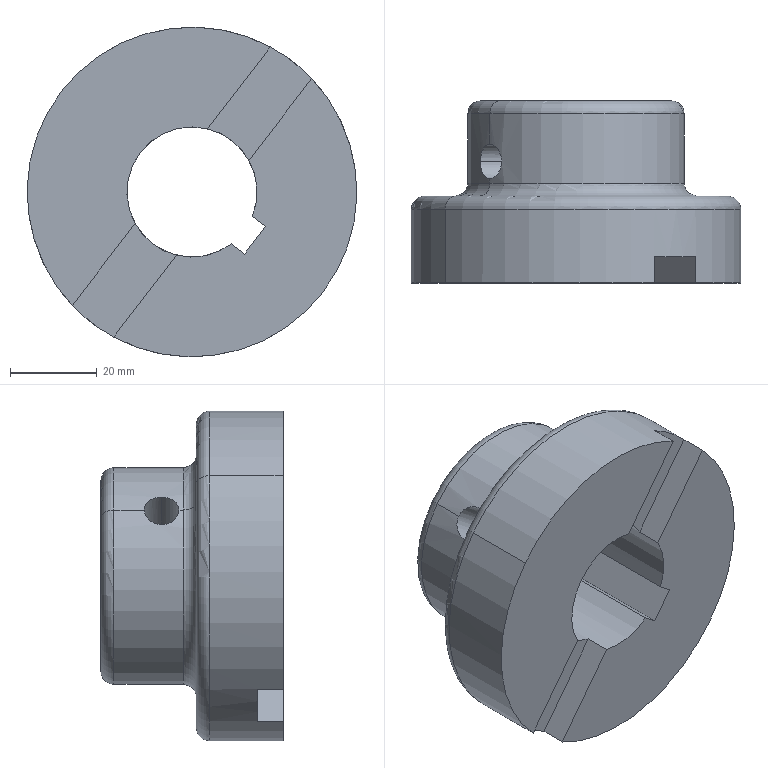Component | SolidWorks | 6-1 | 1 solid | 27 faces | box 76 x 42 x 76 mm | volume 98778 mm3 | plane 13 | cylinder 8 | torus 6 | commonest cylinder face diameters 8 x2 30 x2 50 x2 76 x2
STEP:
#1=COLOUR_RGB('',0.7922,0.8196,0.9333);
#2=FILL_AREA_STYLE_COLOUR('',#1);
#3=FILL_AREA_STYLE('',(#2));
#4=SURFACE_STYLE_FILL_AREA(#3);
#5=SURFACE_SIDE_STYLE('',(#4));
#6=SURFACE_STYLE_USAGE(.BOTH.,#5);
#7=PRESENTATION_STYLE_ASSIGNMENT((#6));
#8=CARTESIAN_POINT('',(-0.5476,-12.882,0.2211));
#9=VERTEX_POINT('',#8);
#10=CARTESIAN_POINT('',(-0.4688,-13.039,0.3591));
#11=VERTEX_POINT('',#10);
#12=CARTESIAN_POINT('',(-0.5476,-12.882,0.2211));
#13=CARTESIAN_POINT('',(-0.5476,-12.892,0.2211));
#14=CARTESIAN_POINT('',(-0.5472,-12.902,0.2221));
#15=CARTESIAN_POINT('',(-0.5456,-12.923,0.226));
#16=CARTESIAN_POINT('',(-0.5444,-12.933,0.2289));
#17=CARTESIAN_POINT('',(-0.5412,-12.952,0.2364));
#18=CARTESIAN_POINT('',(-0.5392,-12.961,0.241));
#19=CARTESIAN_POINT('',(-0.5343,-12.978,0.2517));
#20=CARTESIAN_POINT('',(-0.5314,-12.986,0.2577));
#21=CARTESIAN_POINT('',(-0.5248,-13.,0.2709));
#22=CARTESIAN_POINT('',(-0.521,-13.007,0.2781));
#23=CARTESIAN_POINT('',(-0.5127,-13.018,0.2932));
#24=CARTESIAN_POINT('',(-0.5081,-13.023,0.3011));
#25=CARTESIAN_POINT('',(-0.498,-13.031,0.3175));
#26=CARTESIAN_POINT('',(-0.4926,-13.034,0.3258));
#27=CARTESIAN_POINT('',(-0.4812,-13.038,0.3425));
#28=CARTESIAN_POINT('',(-0.4751,-13.039,0.3509));
#29=CARTESIAN_POINT('',(-0.4688,-13.039,0.3591));
#30=B_SPLINE_CURVE_WITH_KNOTS('',3,(#12,#13,#14,#15,#16,#17,#18,#19,#20,#21,#22,#23,#24,#25,#26,#27,#28,#29),.UNSPECIFIED.,.F.,.F.,(4,2,2,2,2,2,2,2,4),(0.01256,0.01335,0.01413,0.01492,0.0157,0.01649,0.01727,0.01806,0.01884),.UNSPECIFIED.);
#31=EDGE_CURVE('',#9,#11,#30,.T.);
#32=ORIENTED_EDGE('',*,*,#31,.F.);
#33=CARTESIAN_POINT('',(-0.867,-12.882,0.4659));
#34=VERTEX_POINT('',#33);
#35=CARTESIAN_POINT('',(-0.8771,-12.882,0.4736));
#36=DIRECTION('',(-0.7938,0.,0.6082));
#37=VECTOR('',#36,39.37);
#38=LINE('',#35,#37);
#39=EDGE_CURVE('',#9,#34,#38,.T.);
#40=ORIENTED_EDGE('',*,*,#39,.T.);
#41=CARTESIAN_POINT('',(-0.7813,-13.039,0.5986));
#42=VERTEX_POINT('',#41);
#43=CARTESIAN_POINT('',(-0.7813,-13.039,0.5986));
#44=CARTESIAN_POINT('',(-0.7876,-13.039,0.5904));
#45=CARTESIAN_POINT('',(-0.7938,-13.038,0.582));
#46=CARTESIAN_POINT('',(-0.8056,-13.034,0.5656));
#47=CARTESIAN_POINT('',(-0.8112,-13.031,0.5575));
#48=CARTESIAN_POINT('',(-0.8219,-13.023,0.5416));
#49=CARTESIAN_POINT('',(-0.8269,-13.018,0.5339));
#50=CARTESIAN_POINT('',(-0.836,-13.007,0.5195));
#51=CARTESIAN_POINT('',(-0.8402,-13.001,0.5126));
#52=CARTESIAN_POINT('',(-0.8478,-12.986,0.5));
#53=CARTESIAN_POINT('',(-0.8511,-12.978,0.4943));
#54=CARTESIAN_POINT('',(-0.8568,-12.961,0.4844));
#55=CARTESIAN_POINT('',(-0.8593,-12.952,0.48));
#56=CARTESIAN_POINT('',(-0.8631,-12.933,0.473));
#57=CARTESIAN_POINT('',(-0.8646,-12.923,0.4704));
#58=CARTESIAN_POINT('',(-0.8665,-12.903,0.4668));
#59=CARTESIAN_POINT('',(-0.867,-12.892,0.4659));
#60=CARTESIAN_POINT('',(-0.867,-12.882,0.4659));
#61=B_SPLINE_CURVE_WITH_KNOTS('',3,(#43,#44,#45,#46,#47,#48,#49,#50,#51,#52,#53,#54,#55,#56,#57,#58,#59,#60),.UNSPECIFIED.,.F.,.F.,(4,2,2,2,2,2,2,2,4),(0.006264,0.007047,0.00783,0.008613,0.009395,0.01018,0.01096,0.01174,0.01253),.UNSPECIFIED.);
#62=EDGE_CURVE('',#42,#34,#61,.T.);
#63=ORIENTED_EDGE('',*,*,#62,.F.);
#64=CARTESIAN_POINT('',(-0.6755,-12.882,0.7159));
#65=VERTEX_POINT('',#64);
#66=CARTESIAN_POINT('',(-0.6755,-12.882,0.7159));
#67=CARTESIAN_POINT('',(-0.6755,-12.892,0.7159));
#68=CARTESIAN_POINT('',(-0.6762,-12.903,0.7152));
#69=CARTESIAN_POINT('',(-0.6792,-12.923,0.7124));
#70=CARTESIAN_POINT('',(-0.6814,-12.933,0.7102));
#71=CARTESIAN_POINT('',(-0.6872,-12.952,0.7047));
#72=CARTESIAN_POINT('',(-0.6907,-12.961,0.7013));
#73=CARTESIAN_POINT('',(-0.6988,-12.978,0.6931));
#74=CARTESIAN_POINT('',(-0.7035,-12.986,0.6884));
#75=CARTESIAN_POINT('',(-0.7137,-13.001,0.6778));
#76=CARTESIAN_POINT('',(-0.7191,-13.007,0.6721));
#77=CARTESIAN_POINT('',(-0.7308,-13.019,0.6593));
#78=CARTESIAN_POINT('',(-0.737,-13.023,0.6525));
#79=CARTESIAN_POINT('',(-0.7494,-13.031,0.6381));
#80=CARTESIAN_POINT('',(-0.7558,-13.034,0.6305));
#81=CARTESIAN_POINT('',(-0.7687,-13.038,0.6148));
#82=CARTESIAN_POINT('',(-0.7751,-13.039,0.6067));
#83=CARTESIAN_POINT('',(-0.7813,-13.039,0.5986));
#84=B_SPLINE_CURVE_WITH_KNOTS('',3,(#66,#67,#68,#69,#70,#71,#72,#73,#74,#75,#76,#77,#78,#79,#80,#81,#82,#83),.UNSPECIFIED.,.F.,.F.,(4,2,2,2,2,2,2,2,4),(0.,0.0007831,0.001566,0.002349,0.003132,0.003915,0.004698,0.005481,0.006264),.UNSPECIFIED.);
#85=EDGE_CURVE('',#65,#42,#84,.T.);
#86=ORIENTED_EDGE('',*,*,#85,.F.);
#87=CARTESIAN_POINT('',(-0.356,-12.882,0.4712));
#88=VERTEX_POINT('',#87);
#89=CARTESIAN_POINT('',(-0.6855,-12.882,0.7236));
#90=DIRECTION('',(-0.7938,0.,0.6082));
#91=VECTOR('',#90,39.37);
#92=LINE('',#89,#91);
#93=EDGE_CURVE('',#88,#65,#92,.T.);
#94=ORIENTED_EDGE('',*,*,#93,.F.);
#95=CARTESIAN_POINT('',(-0.4688,-13.039,0.3591));
#96=CARTESIAN_POINT('',(-0.4625,-13.039,0.3674));
#97=CARTESIAN_POINT('',(-0.456,-13.038,0.3754));
#98=CARTESIAN_POINT('',(-0.4429,-13.034,0.3908));
#99=CARTESIAN_POINT('',(-0.4361,-13.031,0.3983));
#100=CARTESIAN_POINT('',(-0.423,-13.023,0.4122));
#101=CARTESIAN_POINT('',(-0.4166,-13.019,0.4186));
#102=CARTESIAN_POINT('',(-0.4041,-13.007,0.4307));
#103=CARTESIAN_POINT('',(-0.3982,-13.,0.4362));
#104=CARTESIAN_POINT('',(-0.3872,-12.986,0.446));
#105=CARTESIAN_POINT('',(-0.3821,-12.978,0.4503));
#106=CARTESIAN_POINT('',(-0.373,-12.961,0.4579));
#107=CARTESIAN_POINT('',(-0.3691,-12.952,0.461));
#108=CARTESIAN_POINT('',(-0.3628,-12.933,0.466));
#109=CARTESIAN_POINT('',(-0.3602,-12.923,0.468));
#110=CARTESIAN_POINT('',(-0.3569,-12.903,0.4705));
#111=CARTESIAN_POINT('',(-0.356,-12.892,0.4712));
#112=CARTESIAN_POINT('',(-0.356,-12.882,0.4712));
#113=B_SPLINE_CURVE_WITH_KNOTS('',3,(#95,#96,#97,#98,#99,#100,#101,#102,#103,#104,#105,#106,#107,#108,#109,#110,#111,#112),.UNSPECIFIED.,.F.,.F.,(4,2,2,2,2,2,2,2,4),(0.01884,0.01963,0.02041,0.0212,0.02198,0.02277,0.02355,0.02434,0.02512),.UNSPECIFIED.);
#114=EDGE_CURVE('',#11,#88,#113,.T.);
#115=ORIENTED_EDGE('',*,*,#114,.F.);
#116=EDGE_LOOP('',(#32,#40,#63,#86,#94,#115));
#117=FACE_OUTER_BOUND('',#116,.T.);
#118=CARTESIAN_POINT('',(-0.7813,-12.882,0.5986));
#119=DIRECTION('',(-0.7938,0.,0.6082));
#120=DIRECTION('',(0.6082,0.,0.7938));
#121=AXIS2_PLACEMENT_3D('',#118,#119,#120);
#122=CYLINDRICAL_SURFACE('',#121,0.1575);
#123=ADVANCED_FACE('',(#117),#122,.F.);
#124=CARTESIAN_POINT('',(0.7813,-13.079,-0.5986));
#125=VERTEX_POINT('',#124);
#126=CARTESIAN_POINT('',(-0.7813,-13.079,0.5986));
#127=VERTEX_POINT('',#126);
#128=CARTESIAN_POINT('',(-0.,-13.079,0.));
#129=DIRECTION('',(0.,1.,0.));
#130=DIRECTION('',(-0.7938,0.,0.6082));
#131=AXIS2_PLACEMENT_3D('',#128,#129,#130);
#132=CIRCLE('',#131,0.9843);
#133=EDGE_CURVE('',#125,#127,#132,.T.);
#134=ORIENTED_EDGE('',*,*,#133,.F.);
#135=CARTESIAN_POINT('',(0.8751,-13.197,-0.6704));
#136=VERTEX_POINT('',#135);
#137=CARTESIAN_POINT('',(0.8751,-13.079,-0.6704));
#138=DIRECTION('',(0.6082,0.,0.7938));
#139=DIRECTION('',(0.7938,0.,-0.6082));
#140=AXIS2_PLACEMENT_3D('',#137,#138,#139);
#141=CIRCLE('',#140,0.1181);
#142=EDGE_CURVE('',#125,#136,#141,.T.);
#143=ORIENTED_EDGE('',*,*,#142,.T.);
#144=CARTESIAN_POINT('',(-0.8751,-13.197,0.6704));
#145=VERTEX_POINT('',#144);
#146=CARTESIAN_POINT('',(-0.,-13.197,0.));
#147=DIRECTION('',(0.,-1.,0.));
#148=DIRECTION('',(-0.7938,0.,0.6082));
#149=AXIS2_PLACEMENT_3D('',#146,#147,#148);
#150=CIRCLE('',#149,1.102);
#151=EDGE_CURVE('',#145,#136,#150,.T.);
#152=ORIENTED_EDGE('',*,*,#151,.F.);
#153=CARTESIAN_POINT('',(-0.8751,-13.079,0.6704));
#154=DIRECTION('',(-0.6082,0.,-0.7938));
#155=DIRECTION('',(-0.7938,0.,0.6082));
#156=AXIS2_PLACEMENT_3D('',#153,#154,#155);
#157=CIRCLE('',#156,0.1181);
#158=EDGE_CURVE('',#127,#145,#157,.T.);
#159=ORIENTED_EDGE('',*,*,#158,.F.);
#160=EDGE_LOOP('',(#134,#143,#152,#159));
#161=FACE_OUTER_BOUND('',#160,.T.);
#162=CARTESIAN_POINT('',(-0.,-13.079,0.));
#163=DIRECTION('',(0.,1.,0.));
#164=DIRECTION('',(-0.7938,0.,0.6082));
#165=AXIS2_PLACEMENT_3D('',#162,#163,#164);
#166=TOROIDAL_SURFACE('',#165,1.102,0.1181);
#167=ADVANCED_FACE('',(#161),#166,.F.);
#168=CARTESIAN_POINT('',(0.7813,-12.449,-0.5986));
#169=VERTEX_POINT('',#168);
#170=CARTESIAN_POINT('',(-0.7813,-12.449,0.5986));
#171=VERTEX_POINT('',#170);
#172=CARTESIAN_POINT('',(-0.,-12.449,0.));
#173=DIRECTION('',(0.,-1.,0.));
#174=DIRECTION('',(-0.7938,0.,0.6082));
#175=AXIS2_PLACEMENT_3D('',#172,#173,#174);
#176=CIRCLE('',#175,0.9843);
#177=EDGE_CURVE('',#169,#171,#176,.T.);
#178=ORIENTED_EDGE('',*,*,#177,.F.);
#179=CARTESIAN_POINT('',(0.6876,-12.331,-0.5267));
#180=VERTEX_POINT('',#179);
#181=CARTESIAN_POINT('',(0.6876,-12.449,-0.5267));
#182=DIRECTION('',(0.6082,0.,0.7938));
#183=DIRECTION('',(0.7938,0.,-0.6082));
#184=AXIS2_PLACEMENT_3D('',#181,#182,#183);
#185=CIRCLE('',#184,0.1181);
#186=EDGE_CURVE('',#169,#180,#185,.T.);
#187=ORIENTED_EDGE('',*,*,#186,.T.);
#188=CARTESIAN_POINT('',(-0.6876,-12.331,0.5267));
#189=VERTEX_POINT('',#188);
#190=CARTESIAN_POINT('',(-0.,-12.331,0.));
#191=DIRECTION('',(0.,1.,0.));
#192=DIRECTION('',(-0.7938,0.,0.6082));
#193=AXIS2_PLACEMENT_3D('',#190,#191,#192);
#194=CIRCLE('',#193,0.8661);
#195=EDGE_CURVE('',#189,#180,#194,.T.);
#196=ORIENTED_EDGE('',*,*,#195,.F.);
#197=CARTESIAN_POINT('',(-0.6876,-12.449,0.5267));
#198=DIRECTION('',(-0.6082,0.,-0.7938));
#199=DIRECTION('',(-0.7938,0.,0.6082));
#200=AXIS2_PLACEMENT_3D('',#197,#198,#199);
#201=CIRCLE('',#200,0.1181);
#202=EDGE_CURVE('',#171,#189,#201,.T.);
#203=ORIENTED_EDGE('',*,*,#202,.F.);
#204=EDGE_LOOP('',(#178,#187,#196,#203));
#205=FACE_OUTER_BOUND('',#204,.T.);
#206=CARTESIAN_POINT('',(-0.,-12.449,0.));
#207=DIRECTION('',(0.,1.,0.));
#208=DIRECTION('',(-0.7938,0.,0.6082));
#209=AXIS2_PLACEMENT_3D('',#206,#207,#208);
#210=TOROIDAL_SURFACE('',#209,0.8661,0.1181);
#211=ADVANCED_FACE('',(#205),#210,.T.);
#212=CARTESIAN_POINT('',(1.188,-13.315,-0.9098));
#213=VERTEX_POINT('',#212);
#214=CARTESIAN_POINT('',(-1.188,-13.315,0.9098));
#215=VERTEX_POINT('',#214);
#216=CARTESIAN_POINT('',(-0.,-13.315,0.));
#217=DIRECTION('',(0.,-1.,0.));
#218=DIRECTION('',(-0.7938,0.,0.6082));
#219=AXIS2_PLACEMENT_3D('',#216,#217,#218);
#220=CIRCLE('',#219,1.496);
#221=EDGE_CURVE('',#213,#215,#220,.T.);
#222=ORIENTED_EDGE('',*,*,#221,.F.);
#223=CARTESIAN_POINT('',(1.094,-13.197,-0.838));
#224=VERTEX_POINT('',#223);
#225=CARTESIAN_POINT('',(1.094,-13.315,-0.838));
#226=DIRECTION('',(0.6082,0.,0.7938));
#227=DIRECTION('',(0.7938,0.,-0.6082));
#228=AXIS2_PLACEMENT_3D('',#225,#226,#227);
#229=CIRCLE('',#228,0.1181);
#230=EDGE_CURVE('',#213,#224,#229,.T.);
#231=ORIENTED_EDGE('',*,*,#230,.T.);
#232=CARTESIAN_POINT('',(-1.094,-13.197,0.838));
#233=VERTEX_POINT('',#232);
#234=CARTESIAN_POINT('',(-0.,-13.197,0.));
#235=DIRECTION('',(0.,1.,0.));
#236=DIRECTION('',(-0.7938,0.,0.6082));
#237=AXIS2_PLACEMENT_3D('',#234,#235,#236);
#238=CIRCLE('',#237,1.378);
#239=EDGE_CURVE('',#233,#224,#238,.T.);
#240=ORIENTED_EDGE('',*,*,#239,.F.);
#241=CARTESIAN_POINT('',(-1.094,-13.315,0.838));
#242=DIRECTION('',(-0.6082,0.,-0.7938));
#243=DIRECTION('',(-0.7938,0.,0.6082));
#244=AXIS2_PLACEMENT_3D('',#241,#242,#243);
#245=CIRCLE('',#244,0.1181);
#246=EDGE_CURVE('',#215,#233,#245,.T.);
#247=ORIENTED_EDGE('',*,*,#246,.F.);
#248=EDGE_LOOP('',(#222,#231,#240,#247));
#249=FACE_OUTER_BOUND('',#248,.T.);
#250=CARTESIAN_POINT('',(-0.,-13.315,0.));
#251=DIRECTION('',(0.,1.,0.));
#252=DIRECTION('',(-0.7938,0.,0.6082));
#253=AXIS2_PLACEMENT_3D('',#250,#251,#252);
#254=TOROIDAL_SURFACE('',#253,1.378,0.1181);
#255=ADVANCED_FACE('',(#249),#254,.T.);
#256=CARTESIAN_POINT('',(-0.4688,-13.984,0.3591));
#257=VERTEX_POINT('',#256);
#258=CARTESIAN_POINT('',(0.1416,-13.984,0.5733));
#259=VERTEX_POINT('',#258);
#260=CARTESIAN_POINT('',(-0.,-13.984,0.));
#261=DIRECTION('',(0.,1.,0.));
#262=DIRECTION('',(-0.7938,0.,0.6082));
#263=AXIS2_PLACEMENT_3D('',#260,#261,#262);
#264=CIRCLE('',#263,0.5906);
#265=EDGE_CURVE('',#257,#259,#264,.T.);
#266=ORIENTED_EDGE('',*,*,#265,.F.);
#267=CARTESIAN_POINT('',(-0.4688,-15.047,0.3591));
#268=DIRECTION('',(0.,1.,0.));
#269=VECTOR('',#268,39.37);
#270=LINE('',#267,#269);
#271=EDGE_CURVE('',#257,#11,#270,.T.);
#272=ORIENTED_EDGE('',*,*,#271,.T.);
#273=ORIENTED_EDGE('',*,*,#114,.T.);
#274=CARTESIAN_POINT('',(-0.4688,-12.724,0.3591));
#275=VERTEX_POINT('',#274);
#276=CARTESIAN_POINT('',(-0.356,-12.882,0.4712));
#277=CARTESIAN_POINT('',(-0.356,-12.871,0.4712));
#278=CARTESIAN_POINT('',(-0.3569,-12.861,0.4705));
#279=CARTESIAN_POINT('',(-0.3602,-12.841,0.468));
#280=CARTESIAN_POINT('',(-0.3627,-12.831,0.466));
#281=CARTESIAN_POINT('',(-0.3691,-12.812,0.461));
#282=CARTESIAN_POINT('',(-0.373,-12.803,0.4579));
#283=CARTESIAN_POINT('',(-0.382,-12.786,0.4504));
#284=CARTESIAN_POINT('',(-0.3872,-12.778,0.446));
#285=CARTESIAN_POINT('',(-0.3982,-12.763,0.4362));
#286=CARTESIAN_POINT('',(-0.4041,-12.757,0.4307));
#287=CARTESIAN_POINT('',(-0.4166,-12.745,0.4186));
#288=CARTESIAN_POINT('',(-0.4231,-12.74,0.4121));
#289=CARTESIAN_POINT('',(-0.4361,-12.733,0.3983));
#290=CARTESIAN_POINT('',(-0.4428,-12.729,0.3908));
#291=CARTESIAN_POINT('',(-0.4561,-12.725,0.3753));
#292=CARTESIAN_POINT('',(-0.4625,-12.724,0.3673));
#293=CARTESIAN_POINT('',(-0.4688,-12.724,0.3591));
#294=B_SPLINE_CURVE_WITH_KNOTS('',3,(#276,#277,#278,#279,#280,#281,#282,#283,#284,#285,#286,#287,#288,#289,#290,#291,#292,#293),.UNSPECIFIED.,.F.,.F.,(4,2,2,2,2,2,2,2,4),(0.,0.0007854,0.001571,0.002356,0.003142,0.003927,0.004712,0.005498,0.006283),.UNSPECIFIED.);
#295=EDGE_CURVE('',#88,#275,#294,.T.);
#296=ORIENTED_EDGE('',*,*,#295,.T.);
#297=CARTESIAN_POINT('',(-0.4688,-12.331,0.3591));
#298=VERTEX_POINT('',#297);
#299=CARTESIAN_POINT('',(-0.4688,-15.047,0.3591));
#300=DIRECTION('',(0.,1.,0.));
#301=VECTOR('',#300,39.37);
#302=LINE('',#299,#301);
#303=EDGE_CURVE('',#275,#298,#302,.T.);
#304=ORIENTED_EDGE('',*,*,#303,.T.);
#305=CARTESIAN_POINT('',(0.5476,-12.331,-0.2211));
#306=VERTEX_POINT('',#305);
#307=CARTESIAN_POINT('',(-0.,-12.331,0.));
#308=DIRECTION('',(0.,1.,0.));
#309=DIRECTION('',(-0.7938,0.,0.6082));
#310=AXIS2_PLACEMENT_3D('',#307,#308,#309);
#311=CIRCLE('',#310,0.5906);
#312=EDGE_CURVE('',#298,#306,#311,.T.);
#313=ORIENTED_EDGE('',*,*,#312,.T.);
#314=CARTESIAN_POINT('',(0.5476,-13.984,-0.2211));
#315=VERTEX_POINT('',#314);
#316=CARTESIAN_POINT('',(0.5476,-15.047,-0.2211));
#317=DIRECTION('',(0.,1.,0.));
#318=VECTOR('',#317,39.37);
#319=LINE('',#316,#318);
#320=EDGE_CURVE('',#315,#306,#319,.T.);
#321=ORIENTED_EDGE('',*,*,#320,.F.);
#322=CARTESIAN_POINT('',(0.5167,-13.984,0.286));
#323=VERTEX_POINT('',#322);
#324=CARTESIAN_POINT('',(-0.,-13.984,0.));
#325=DIRECTION('',(0.,1.,0.));
#326=DIRECTION('',(-0.7938,0.,0.6082));
#327=AXIS2_PLACEMENT_3D('',#324,#325,#326);
#328=CIRCLE('',#327,0.5906);
#329=EDGE_CURVE('',#323,#315,#328,.T.);
#330=ORIENTED_EDGE('',*,*,#329,.F.);
#331=CARTESIAN_POINT('',(0.5167,-13.748,0.286));
#332=VERTEX_POINT('',#331);
#333=CARTESIAN_POINT('',(0.5167,-15.047,0.286));
#334=DIRECTION('',(0.,1.,0.));
#335=VECTOR('',#334,39.37);
#336=LINE('',#333,#335);
#337=EDGE_CURVE('',#323,#332,#336,.T.);
#338=ORIENTED_EDGE('',*,*,#337,.T.);
#339=CARTESIAN_POINT('',(0.1416,-13.748,0.5733));
#340=VERTEX_POINT('',#339);
#341=CARTESIAN_POINT('',(-0.,-13.748,0.));
#342=DIRECTION('',(0.,-1.,0.));
#343=DIRECTION('',(-0.7938,0.,0.6082));
#344=AXIS2_PLACEMENT_3D('',#341,#342,#343);
#345=CIRCLE('',#344,0.5906);
#346=EDGE_CURVE('',#332,#340,#345,.T.);
#347=ORIENTED_EDGE('',*,*,#346,.T.);
#348=CARTESIAN_POINT('',(0.1416,-15.047,0.5733));
#349=DIRECTION('',(0.,-1.,0.));
#350=VECTOR('',#349,39.37);
#351=LINE('',#348,#350);
#352=EDGE_CURVE('',#340,#259,#351,.T.);
#353=ORIENTED_EDGE('',*,*,#352,.T.);
#354=EDGE_LOOP('',(#266,#272,#273,#296,#304,#313,#321,#330,#338,#347,#353));
#355=FACE_OUTER_BOUND('',#354,.T.);
#356=CARTESIAN_POINT('',(-0.,-15.047,0.));
#357=DIRECTION('',(0.,1.,0.));
#358=DIRECTION('',(-0.7938,0.,0.6082));
#359=AXIS2_PLACEMENT_3D('',#356,#357,#358);
#360=CYLINDRICAL_SURFACE('',#359,0.5906);
#361=ADVANCED_FACE('',(#355),#360,.F.);
#362=ORIENTED_EDGE('',*,*,#177,.T.);
#363=CARTESIAN_POINT('',(-0.7813,-12.724,0.5986));
#364=VERTEX_POINT('',#363);
#365=CARTESIAN_POINT('',(-0.7813,-12.331,0.5986));
#366=DIRECTION('',(0.,-1.,0.));
#367=VECTOR('',#366,39.37);
#368=LINE('',#365,#367);
#369=EDGE_CURVE('',#171,#364,#368,.T.);
#370=ORIENTED_EDGE('',*,*,#369,.T.);
#371=CARTESIAN_POINT('',(-0.7813,-12.724,0.5986));
#372=CARTESIAN_POINT('',(-0.775,-12.724,0.6068));
#373=CARTESIAN_POINT('',(-0.7686,-12.725,0.6149));
#374=CARTESIAN_POINT('',(-0.7559,-12.729,0.6305));
#375=CARTESIAN_POINT('',(-0.7494,-12.732,0.6381));
#376=CARTESIAN_POINT('',(-0.7369,-12.74,0.6525));
#377=CARTESIAN_POINT('',(-0.7309,-12.745,0.6593));
#378=CARTESIAN_POINT('',(-0.7192,-12.757,0.6719));
#379=CARTESIAN_POINT('',(-0.7137,-12.763,0.6779));
#380=CARTESIAN_POINT('',(-0.7035,-12.778,0.6884));
#381=CARTESIAN_POINT('',(-0.6989,-12.786,0.693));
#382=CARTESIAN_POINT('',(-0.6907,-12.803,0.7012));
#383=CARTESIAN_POINT('',(-0.6872,-12.812,0.7047));
#384=CARTESIAN_POINT('',(-0.6815,-12.831,0.7102));
#385=CARTESIAN_POINT('',(-0.6792,-12.841,0.7123));
#386=CARTESIAN_POINT('',(-0.6762,-12.861,0.7152));
#387=CARTESIAN_POINT('',(-0.6755,-12.871,0.7159));
#388=CARTESIAN_POINT('',(-0.6755,-12.882,0.7159));
#389=B_SPLINE_CURVE_WITH_KNOTS('',3,(#371,#372,#373,#374,#375,#376,#377,#378,#379,#380,#381,#382,#383,#384,#385,#386,#387,#388),.UNSPECIFIED.,.F.,.F.,(4,2,2,2,2,2,2,2,4),(0.01879,0.01957,0.02035,0.02114,0.02192,0.0227,0.02348,0.02427,0.02505),.UNSPECIFIED.);
#390=EDGE_CURVE('',#364,#65,#389,.T.);
#391=ORIENTED_EDGE('',*,*,#390,.T.);
#392=ORIENTED_EDGE('',*,*,#85,.T.);
#393=CARTESIAN_POINT('',(-0.7813,-12.331,0.5986));
#394=DIRECTION('',(0.,-1.,0.));
#395=VECTOR('',#394,39.37);
#396=LINE('',#393,#395);
#397=EDGE_CURVE('',#42,#127,#396,.T.);
#398=ORIENTED_EDGE('',*,*,#397,.T.);
#399=CARTESIAN_POINT('',(-0.,-13.079,0.));
#400=DIRECTION('',(0.,1.,0.));
#401=DIRECTION('',(-0.7938,0.,0.6082));
#402=AXIS2_PLACEMENT_3D('',#399,#400,#401);
#403=CIRCLE('',#402,0.9843);
#404=EDGE_CURVE('',#127,#125,#403,.T.);
#405=ORIENTED_EDGE('',*,*,#404,.T.);
#406=CARTESIAN_POINT('',(0.7813,-12.331,-0.5986));
#407=DIRECTION('',(0.,-1.,0.));
#408=VECTOR('',#407,39.37);
#409=LINE('',#406,#408);
#410=EDGE_CURVE('',#169,#125,#409,.T.);
#411=ORIENTED_EDGE('',*,*,#410,.F.);
#412=EDGE_LOOP('',(#362,#370,#391,#392,#398,#405,#411));
#413=FACE_OUTER_BOUND('',#412,.T.);
#414=CARTESIAN_POINT('',(-0.,-12.331,0.));
#415=DIRECTION('',(0.,-1.,0.));
#416=DIRECTION('',(0.7938,0.,-0.6082));
#417=AXIS2_PLACEMENT_3D('',#414,#415,#416);
#418=CYLINDRICAL_SURFACE('',#417,0.9843);
#419=ADVANCED_FACE('',(#413),#418,.T.);
#420=ORIENTED_EDGE('',*,*,#221,.T.);
#421=CARTESIAN_POINT('',(-1.188,-13.984,0.9098));
#422=VERTEX_POINT('',#421);
#423=CARTESIAN_POINT('',(-1.188,-13.197,0.9098));
#424=DIRECTION('',(0.,-1.,0.));
#425=VECTOR('',#424,39.37);
#426=LINE('',#423,#425);
#427=EDGE_CURVE('',#215,#422,#426,.T.);
#428=ORIENTED_EDGE('',*,*,#427,.T.);
#429=CARTESIAN_POINT('',(0.7109,-13.984,1.316));
#430=VERTEX_POINT('',#429);
#431=CARTESIAN_POINT('',(-0.,-13.984,0.));
#432=DIRECTION('',(0.,1.,0.));
#433=DIRECTION('',(-0.7938,0.,0.6082));
#434=AXIS2_PLACEMENT_3D('',#431,#432,#433);
#435=CIRCLE('',#434,1.496);
#436=EDGE_CURVE('',#422,#430,#435,.T.);
#437=ORIENTED_EDGE('',*,*,#436,.T.);
#438=CARTESIAN_POINT('',(0.7109,-13.748,1.316));
#439=VERTEX_POINT('',#438);
#440=CARTESIAN_POINT('',(0.7109,-13.197,1.316));
#441=DIRECTION('',(0.,1.,0.));
#442=VECTOR('',#441,39.37);
#443=LINE('',#440,#442);
#444=EDGE_CURVE('',#430,#439,#443,.T.);
#445=ORIENTED_EDGE('',*,*,#444,.T.);
#446=CARTESIAN_POINT('',(1.086,-13.748,1.029));
#447=VERTEX_POINT('',#446);
#448=CARTESIAN_POINT('',(-0.,-13.748,0.));
#449=DIRECTION('',(0.,1.,0.));
#450=DIRECTION('',(-0.7938,0.,0.6082));
#451=AXIS2_PLACEMENT_3D('',#448,#449,#450);
#452=CIRCLE('',#451,1.496);
#453=EDGE_CURVE('',#439,#447,#452,.T.);
#454=ORIENTED_EDGE('',*,*,#453,.T.);
#455=CARTESIAN_POINT('',(1.086,-13.984,1.029));
#456=VERTEX_POINT('',#455);
#457=CARTESIAN_POINT('',(1.086,-13.197,1.029));
#458=DIRECTION('',(0.,-1.,0.));
#459=VECTOR('',#458,39.37);
#460=LINE('',#457,#459);
#461=EDGE_CURVE('',#447,#456,#460,.T.);
#462=ORIENTED_EDGE('',*,*,#461,.T.);
#463=CARTESIAN_POINT('',(1.188,-13.984,-0.9098));
#464=VERTEX_POINT('',#463);
#465=CARTESIAN_POINT('',(-0.,-13.984,0.));
#466=DIRECTION('',(0.,1.,0.));
#467=DIRECTION('',(-0.7938,0.,0.6082));
#468=AXIS2_PLACEMENT_3D('',#465,#466,#467);
#469=CIRCLE('',#468,1.496);
#470=EDGE_CURVE('',#456,#464,#469,.T.);
#471=ORIENTED_EDGE('',*,*,#470,.T.);
#472=CARTESIAN_POINT('',(1.188,-13.197,-0.9098));
#473=DIRECTION('',(0.,-1.,0.));
#474=VECTOR('',#473,39.37);
#475=LINE('',#472,#474);
#476=EDGE_CURVE('',#213,#464,#475,.T.);
#477=ORIENTED_EDGE('',*,*,#476,.F.);
#478=EDGE_LOOP('',(#420,#428,#437,#445,#454,#462,#471,#477));
#479=FACE_OUTER_BOUND('',#478,.T.);
#480=CARTESIAN_POINT('',(-0.,-13.197,0.));
#481=DIRECTION('',(0.,-1.,0.));
#482=DIRECTION('',(0.7938,0.,-0.6082));
#483=AXIS2_PLACEMENT_3D('',#480,#481,#482);
#484=CYLINDRICAL_SURFACE('',#483,1.496);
#485=ADVANCED_FACE('',(#479),#484,.T.);
#486=CARTESIAN_POINT('',(-1.086,-13.984,-1.029));
#487=VERTEX_POINT('',#486);
#488=CARTESIAN_POINT('',(-0.,-13.984,0.));
#489=DIRECTION('',(0.,1.,0.));
#490=DIRECTION('',(-0.7938,0.,0.6082));
#491=AXIS2_PLACEMENT_3D('',#488,#489,#490);
#492=CIRCLE('',#491,1.496);
#493=EDGE_CURVE('',#487,#422,#492,.T.);
#494=ORIENTED_EDGE('',*,*,#493,.F.);
#495=CARTESIAN_POINT('',(-0.5167,-13.984,-0.286));
#496=VERTEX_POINT('',#495);
#497=CARTESIAN_POINT('',(0.8647,-13.984,1.517));
#498=DIRECTION('',(-0.6082,0.,-0.7938));
#499=VECTOR('',#498,39.37);
#500=LINE('',#497,#499);
#501=EDGE_CURVE('',#496,#487,#500,.T.);
#502=ORIENTED_EDGE('',*,*,#501,.F.);
#503=CARTESIAN_POINT('',(-0.,-13.984,0.));
#504=DIRECTION('',(0.,1.,0.));
#505=DIRECTION('',(-0.7938,0.,0.6082));
#506=AXIS2_PLACEMENT_3D('',#503,#504,#505);
#507=CIRCLE('',#506,0.5906);
#508=EDGE_CURVE('',#496,#257,#507,.T.);
#509=ORIENTED_EDGE('',*,*,#508,.T.);
#510=ORIENTED_EDGE('',*,*,#265,.T.);
#511=CARTESIAN_POINT('',(0.8647,-13.984,1.517));
#512=DIRECTION('',(-0.6082,0.,-0.7938));
#513=VECTOR('',#512,39.37);
#514=LINE('',#511,#513);
#515=EDGE_CURVE('',#430,#259,#514,.T.);
#516=ORIENTED_EDGE('',*,*,#515,.F.);
#517=ORIENTED_EDGE('',*,*,#436,.F.);
#518=EDGE_LOOP('',(#494,#502,#509,#510,#516,#517));
#519=FACE_OUTER_BOUND('',#518,.T.);
#520=CARTESIAN_POINT('',(-0.,-13.984,0.));
#521=DIRECTION('',(0.,1.,0.));
#522=DIRECTION('',(-0.7938,0.,0.6082));
#523=AXIS2_PLACEMENT_3D('',#520,#521,#522);
#524=PLANE('',#523);
#525=ADVANCED_FACE('',(#519),#524,.F.);
#526=ORIENTED_EDGE('',*,*,#427,.F.);
#527=CARTESIAN_POINT('',(-0.,-13.315,0.));
#528=DIRECTION('',(0.,-1.,0.));
#529=DIRECTION('',(-0.7938,0.,0.6082));
#530=AXIS2_PLACEMENT_3D('',#527,#528,#529);
#531=CIRCLE('',#530,1.496);
#532=EDGE_CURVE('',#215,#213,#531,.T.);
#533=ORIENTED_EDGE('',*,*,#532,.T.);
#534=ORIENTED_EDGE('',*,*,#476,.T.);
#535=CARTESIAN_POINT('',(-0.7109,-13.984,-1.316));
#536=VERTEX_POINT('',#535);
#537=CARTESIAN_POINT('',(-0.,-13.984,0.));
#538=DIRECTION('',(0.,1.,0.));
#539=DIRECTION('',(-0.7938,0.,0.6082));
#540=AXIS2_PLACEMENT_3D('',#537,#538,#539);
#541=CIRCLE('',#540,1.496);
#542=EDGE_CURVE('',#464,#536,#541,.T.);
#543=ORIENTED_EDGE('',*,*,#542,.T.);
#544=CARTESIAN_POINT('',(-0.7109,-13.748,-1.316));
#545=VERTEX_POINT('',#544);
#546=CARTESIAN_POINT('',(-0.7109,-13.197,-1.316));
#547=DIRECTION('',(0.,1.,0.));
#548=VECTOR('',#547,39.37);
#549=LINE('',#546,#548);
#550=EDGE_CURVE('',#536,#545,#549,.T.);
#551=ORIENTED_EDGE('',*,*,#550,.T.);
#552=CARTESIAN_POINT('',(-1.086,-13.748,-1.029));
#553=VERTEX_POINT('',#552);
#554=CARTESIAN_POINT('',(-0.,-13.748,0.));
#555=DIRECTION('',(0.,1.,0.));
#556=DIRECTION('',(-0.7938,0.,0.6082));
#557=AXIS2_PLACEMENT_3D('',#554,#555,#556);
#558=CIRCLE('',#557,1.496);
#559=EDGE_CURVE('',#545,#553,#558,.T.);
#560=ORIENTED_EDGE('',*,*,#559,.T.);
#561=CARTESIAN_POINT('',(-1.086,-13.197,-1.029));
#562=DIRECTION('',(0.,-1.,0.));
#563=VECTOR('',#562,39.37);
#564=LINE('',#561,#563);
#565=EDGE_CURVE('',#553,#487,#564,.T.);
#566=ORIENTED_EDGE('',*,*,#565,.T.);
#567=ORIENTED_EDGE('',*,*,#493,.T.);
#568=EDGE_LOOP('',(#526,#533,#534,#543,#551,#560,#566,#567));
#569=FACE_OUTER_BOUND('',#568,.T.);
#570=CARTESIAN_POINT('',(-0.,-13.197,0.));
#571=DIRECTION('',(0.,-1.,0.));
#572=DIRECTION('',(0.7938,0.,-0.6082));
#573=AXIS2_PLACEMENT_3D('',#570,#571,#572);
#574=CYLINDRICAL_SURFACE('',#573,1.496);
#575=ADVANCED_FACE('',(#569),#574,.T.);
#576=ORIENTED_EDGE('',*,*,#151,.T.);
#577=CARTESIAN_POINT('',(-0.,-13.197,0.));
#578=DIRECTION('',(0.,-1.,0.));
#579=DIRECTION('',(-0.7938,0.,0.6082));
#580=AXIS2_PLACEMENT_3D('',#577,#578,#579);
#581=CIRCLE('',#580,1.102);
#582=EDGE_CURVE('',#136,#145,#581,.T.);
#583=ORIENTED_EDGE('',*,*,#582,.T.);
#584=EDGE_LOOP('',(#576,#583));
#585=FACE_BOUND('',#584,.T.);
#586=ORIENTED_EDGE('',*,*,#239,.T.);
#587=CARTESIAN_POINT('',(-0.,-13.197,0.));
#588=DIRECTION('',(0.,1.,0.));
#589=DIRECTION('',(-0.7938,0.,0.6082));
#590=AXIS2_PLACEMENT_3D('',#587,#588,#589);
#591=CIRCLE('',#590,1.378);
#592=EDGE_CURVE('',#224,#233,#591,.T.);
#593=ORIENTED_EDGE('',*,*,#592,.T.);
#594=EDGE_LOOP('',(#586,#593));
#595=FACE_OUTER_BOUND('',#594,.T.);
#596=CARTESIAN_POINT('',(-0.,-13.197,0.));
#597=DIRECTION('',(0.,1.,0.));
#598=DIRECTION('',(-0.7938,0.,0.6082));
#599=AXIS2_PLACEMENT_3D('',#596,#597,#598);
#600=PLANE('',#599);
#601=ADVANCED_FACE('',(#585,#595),#600,.T.);
#602=ORIENTED_EDGE('',*,*,#470,.F.);
#603=CARTESIAN_POINT('',(1.24,-13.984,1.23));
#604=DIRECTION('',(0.6082,0.,0.7938));
#605=VECTOR('',#604,39.37);
#606=LINE('',#603,#605);
#607=EDGE_CURVE('',#323,#456,#606,.T.);
#608=ORIENTED_EDGE('',*,*,#607,.F.);
#609=ORIENTED_EDGE('',*,*,#329,.T.);
#610=CARTESIAN_POINT('',(0.6677,-13.984,-0.3131));
#611=VERTEX_POINT('',#610);
#612=CARTESIAN_POINT('',(0.09577,-13.984,0.125));
#613=DIRECTION('',(0.7938,0.,-0.6082));
#614=VECTOR('',#613,39.37);
#615=LINE('',#612,#614);
#616=EDGE_CURVE('',#315,#611,#615,.T.);
#617=ORIENTED_EDGE('',*,*,#616,.T.);
#618=CARTESIAN_POINT('',(0.4762,-13.984,-0.5632));
#619=VERTEX_POINT('',#618);
#620=CARTESIAN_POINT('',(0.5719,-13.984,-0.4382));
#621=DIRECTION('',(-0.6082,0.,-0.7938));
#622=VECTOR('',#621,39.37);
#623=LINE('',#620,#622);
#624=EDGE_CURVE('',#611,#619,#623,.T.);
#625=ORIENTED_EDGE('',*,*,#624,.T.);
#626=CARTESIAN_POINT('',(0.356,-13.984,-0.4712));
#627=VERTEX_POINT('',#626);
#628=CARTESIAN_POINT('',(-0.09577,-13.984,-0.125));
#629=DIRECTION('',(-0.7938,0.,0.6082));
#630=VECTOR('',#629,39.37);
#631=LINE('',#628,#630);
#632=EDGE_CURVE('',#619,#627,#631,.T.);
#633=ORIENTED_EDGE('',*,*,#632,.T.);
#634=CARTESIAN_POINT('',(-0.1416,-13.984,-0.5733));
#635=VERTEX_POINT('',#634);
#636=CARTESIAN_POINT('',(-0.,-13.984,0.));
#637=DIRECTION('',(0.,1.,0.));
#638=DIRECTION('',(-0.7938,0.,0.6082));
#639=AXIS2_PLACEMENT_3D('',#636,#637,#638);
#640=CIRCLE('',#639,0.5906);
#641=EDGE_CURVE('',#627,#635,#640,.T.);
#642=ORIENTED_EDGE('',*,*,#641,.T.);
#643=CARTESIAN_POINT('',(1.24,-13.984,1.23));
#644=DIRECTION('',(0.6082,0.,0.7938));
#645=VECTOR('',#644,39.37);
#646=LINE('',#643,#645);
#647=EDGE_CURVE('',#536,#635,#646,.T.);
#648=ORIENTED_EDGE('',*,*,#647,.F.);
#649=ORIENTED_EDGE('',*,*,#542,.F.);
#650=EDGE_LOOP('',(#602,#608,#609,#617,#625,#633,#642,#648,#649));
#651=FACE_OUTER_BOUND('',#650,.T.);
#652=CARTESIAN_POINT('',(-0.,-13.984,0.));
#653=DIRECTION('',(0.,1.,0.));
#654=DIRECTION('',(-0.7938,0.,0.6082));
#655=AXIS2_PLACEMENT_3D('',#652,#653,#654);
#656=PLANE('',#655);
#657=ADVANCED_FACE('',(#651),#656,.F.);
#658=ORIENTED_EDGE('',*,*,#369,.F.);
#659=CARTESIAN_POINT('',(-0.,-12.449,0.));
#660=DIRECTION('',(0.,-1.,0.));
#661=DIRECTION('',(-0.7938,0.,0.6082));
#662=AXIS2_PLACEMENT_3D('',#659,#660,#661);
#663=CIRCLE('',#662,0.9843);
#664=EDGE_CURVE('',#171,#169,#663,.T.);
#665=ORIENTED_EDGE('',*,*,#664,.T.);
#666=ORIENTED_EDGE('',*,*,#410,.T.);
#667=ORIENTED_EDGE('',*,*,#133,.T.);
#668=ORIENTED_EDGE('',*,*,#397,.F.);
#669=ORIENTED_EDGE('',*,*,#62,.T.);
#670=CARTESIAN_POINT('',(-0.867,-12.882,0.4659));
#671=CARTESIAN_POINT('',(-0.867,-12.872,0.4659));
#672=CARTESIAN_POINT('',(-0.8665,-12.861,0.4667));
#673=CARTESIAN_POINT('',(-0.8646,-12.841,0.4704));
#674=CARTESIAN_POINT('',(-0.8631,-12.831,0.473));
#675=CARTESIAN_POINT('',(-0.8593,-12.812,0.48));
#676=CARTESIAN_POINT('',(-0.8569,-12.803,0.4843));
#677=CARTESIAN_POINT('',(-0.8511,-12.786,0.4944));
#678=CARTESIAN_POINT('',(-0.8478,-12.778,0.5));
#679=CARTESIAN_POINT('',(-0.8403,-12.763,0.5126));
#680=CARTESIAN_POINT('',(-0.836,-12.757,0.5195));
#681=CARTESIAN_POINT('',(-0.8268,-12.745,0.534));
#682=CARTESIAN_POINT('',(-0.8219,-12.74,0.5416));
#683=CARTESIAN_POINT('',(-0.8112,-12.732,0.5575));
#684=CARTESIAN_POINT('',(-0.8055,-12.729,0.5657));
#685=CARTESIAN_POINT('',(-0.7938,-12.725,0.582));
#686=CARTESIAN_POINT('',(-0.7876,-12.724,0.5903));
#687=CARTESIAN_POINT('',(-0.7813,-12.724,0.5986));
#688=B_SPLINE_CURVE_WITH_KNOTS('',3,(#670,#671,#672,#673,#674,#675,#676,#677,#678,#679,#680,#681,#682,#683,#684,#685,#686,#687),.UNSPECIFIED.,.F.,.F.,(4,2,2,2,2,2,2,2,4),(0.01253,0.01331,0.01409,0.01487,0.01566,0.01644,0.01722,0.01801,0.01879),.UNSPECIFIED.);
#689=EDGE_CURVE('',#34,#364,#688,.T.);
#690=ORIENTED_EDGE('',*,*,#689,.T.);
#691=EDGE_LOOP('',(#658,#665,#666,#667,#668,#669,#690));
#692=FACE_OUTER_BOUND('',#691,.T.);
#693=CARTESIAN_POINT('',(-0.,-12.331,0.));
#694=DIRECTION('',(0.,-1.,0.));
#695=DIRECTION('',(0.7938,0.,-0.6082));
#696=AXIS2_PLACEMENT_3D('',#693,#694,#695);
#697=CYLINDRICAL_SURFACE('',#696,0.9843);
#698=ADVANCED_FACE('',(#692),#697,.T.);
#699=ORIENTED_EDGE('',*,*,#195,.T.);
#700=CARTESIAN_POINT('',(-0.,-12.331,0.));
#701=DIRECTION('',(0.,1.,0.));
#702=DIRECTION('',(-0.7938,0.,0.6082));
#703=AXIS2_PLACEMENT_3D('',#700,#701,#702);
#704=CIRCLE('',#703,0.8661);
#705=EDGE_CURVE('',#180,#189,#704,.T.);
#706=ORIENTED_EDGE('',*,*,#705,.T.);
#707=EDGE_LOOP('',(#699,#706));
#708=FACE_OUTER_BOUND('',#707,.T.);
#709=CARTESIAN_POINT('',(0.4762,-12.331,-0.5632));
#710=VERTEX_POINT('',#709);
#711=CARTESIAN_POINT('',(0.356,-12.331,-0.4712));
#712=VERTEX_POINT('',#711);
#713=CARTESIAN_POINT('',(0.4762,-12.331,-0.5632));
#714=DIRECTION('',(-0.7938,0.,0.6082));
#715=VECTOR('',#714,39.37);
#716=LINE('',#713,#715);
#717=EDGE_CURVE('',#710,#712,#716,.T.);
#718=ORIENTED_EDGE('',*,*,#717,.F.);
#719=CARTESIAN_POINT('',(0.6677,-12.331,-0.3131));
#720=VERTEX_POINT('',#719);
#721=CARTESIAN_POINT('',(0.6677,-12.331,-0.3131));
#722=DIRECTION('',(-0.6082,0.,-0.7938));
#723=VECTOR('',#722,39.37);
#724=LINE('',#721,#723);
#725=EDGE_CURVE('',#720,#710,#724,.T.);
#726=ORIENTED_EDGE('',*,*,#725,.F.);
#727=CARTESIAN_POINT('',(0.6677,-12.331,-0.3131));
#728=DIRECTION('',(0.7938,0.,-0.6082));
#729=VECTOR('',#728,39.37);
#730=LINE('',#727,#729);
#731=EDGE_CURVE('',#306,#720,#730,.T.);
#732=ORIENTED_EDGE('',*,*,#731,.F.);
#733=ORIENTED_EDGE('',*,*,#312,.F.);
#734=CARTESIAN_POINT('',(-0.,-12.331,0.));
#735=DIRECTION('',(0.,1.,0.));
#736=DIRECTION('',(-0.7938,0.,0.6082));
#737=AXIS2_PLACEMENT_3D('',#734,#735,#736);
#738=CIRCLE('',#737,0.5906);
#739=EDGE_CURVE('',#712,#298,#738,.T.);
#740=ORIENTED_EDGE('',*,*,#739,.F.);
#741=EDGE_LOOP('',(#718,#726,#732,#733,#740));
#742=FACE_BOUND('',#741,.T.);
#743=CARTESIAN_POINT('',(-0.,-12.331,0.));
#744=DIRECTION('',(0.,1.,0.));
#745=DIRECTION('',(-0.7938,0.,0.6082));
#746=AXIS2_PLACEMENT_3D('',#743,#744,#745);
#747=PLANE('',#746);
#748=ADVANCED_FACE('',(#708,#742),#747,.T.);
#749=CARTESIAN_POINT('',(0.4762,-15.047,-0.5632));
#750=DIRECTION('',(0.,1.,0.));
#751=VECTOR('',#750,39.37);
#752=LINE('',#749,#751);
#753=EDGE_CURVE('',#619,#710,#752,.T.);
#754=ORIENTED_EDGE('',*,*,#753,.T.);
#755=ORIENTED_EDGE('',*,*,#717,.T.);
#756=CARTESIAN_POINT('',(0.356,-15.047,-0.4712));
#757=DIRECTION('',(0.,1.,0.));
#758=VECTOR('',#757,39.37);
#759=LINE('',#756,#758);
#760=EDGE_CURVE('',#627,#712,#759,.T.);
#761=ORIENTED_EDGE('',*,*,#760,.F.);
#762=ORIENTED_EDGE('',*,*,#632,.F.);
#763=EDGE_LOOP('',(#754,#755,#761,#762));
#764=FACE_OUTER_BOUND('',#763,.T.);
#765=CARTESIAN_POINT('',(0.4762,-15.047,-0.5632));
#766=DIRECTION('',(-0.6082,0.,-0.7938));
#767=DIRECTION('',(-0.7938,0.,0.6082));
#768=AXIS2_PLACEMENT_3D('',#765,#766,#767);
#769=PLANE('',#768);
#770=ADVANCED_FACE('',(#764),#769,.F.);
#771=CARTESIAN_POINT('',(0.6677,-15.047,-0.3131));
#772=DIRECTION('',(0.,1.,0.));
#773=VECTOR('',#772,39.37);
#774=LINE('',#771,#773);
#775=EDGE_CURVE('',#611,#720,#774,.T.);
#776=ORIENTED_EDGE('',*,*,#775,.T.);
#777=ORIENTED_EDGE('',*,*,#725,.T.);
#778=ORIENTED_EDGE('',*,*,#753,.F.);
#779=ORIENTED_EDGE('',*,*,#624,.F.);
#780=EDGE_LOOP('',(#776,#777,#778,#779));
#781=FACE_OUTER_BOUND('',#780,.T.);
#782=CARTESIAN_POINT('',(0.6677,-15.047,-0.3131));
#783=DIRECTION('',(0.7938,0.,-0.6082));
#784=DIRECTION('',(-0.6082,0.,-0.7938));
#785=AXIS2_PLACEMENT_3D('',#782,#783,#784);
#786=PLANE('',#785);
#787=ADVANCED_FACE('',(#781),#786,.F.);
#788=ORIENTED_EDGE('',*,*,#320,.T.);
#789=ORIENTED_EDGE('',*,*,#731,.T.);
#790=ORIENTED_EDGE('',*,*,#775,.F.);
#791=ORIENTED_EDGE('',*,*,#616,.F.);
#792=EDGE_LOOP('',(#788,#789,#790,#791));
#793=FACE_OUTER_BOUND('',#792,.T.);
#794=CARTESIAN_POINT('',(0.6677,-15.047,-0.3131));
#795=DIRECTION('',(0.6082,0.,0.7938));
#796=DIRECTION('',(0.7938,0.,-0.6082));
#797=AXIS2_PLACEMENT_3D('',#794,#795,#796);
#798=PLANE('',#797);
#799=ADVANCED_FACE('',(#793),#798,.F.);
#800=ORIENTED_EDGE('',*,*,#271,.F.);
#801=ORIENTED_EDGE('',*,*,#508,.F.);
#802=CARTESIAN_POINT('',(-0.5167,-13.748,-0.286));
#803=VERTEX_POINT('',#802);
#804=CARTESIAN_POINT('',(-0.5167,-15.047,-0.286));
#805=DIRECTION('',(0.,1.,0.));
#806=VECTOR('',#805,39.37);
#807=LINE('',#804,#806);
#808=EDGE_CURVE('',#496,#803,#807,.T.);
#809=ORIENTED_EDGE('',*,*,#808,.T.);
#810=CARTESIAN_POINT('',(-0.1416,-13.748,-0.5733));
#811=VERTEX_POINT('',#810);
#812=CARTESIAN_POINT('',(-0.,-13.748,0.));
#813=DIRECTION('',(0.,-1.,0.));
#814=DIRECTION('',(-0.7938,0.,0.6082));
#815=AXIS2_PLACEMENT_3D('',#812,#813,#814);
#816=CIRCLE('',#815,0.5906);
#817=EDGE_CURVE('',#803,#811,#816,.T.);
#818=ORIENTED_EDGE('',*,*,#817,.T.);
#819=CARTESIAN_POINT('',(-0.1416,-15.047,-0.5733));
#820=DIRECTION('',(0.,-1.,0.));
#821=VECTOR('',#820,39.37);
#822=LINE('',#819,#821);
#823=EDGE_CURVE('',#811,#635,#822,.T.);
#824=ORIENTED_EDGE('',*,*,#823,.T.);
#825=ORIENTED_EDGE('',*,*,#641,.F.);
#826=ORIENTED_EDGE('',*,*,#760,.T.);
#827=ORIENTED_EDGE('',*,*,#739,.T.);
#828=ORIENTED_EDGE('',*,*,#303,.F.);
#829=CARTESIAN_POINT('',(-0.4688,-12.724,0.3591));
#830=CARTESIAN_POINT('',(-0.4751,-12.724,0.351));
#831=CARTESIAN_POINT('',(-0.4812,-12.725,0.3425));
#832=CARTESIAN_POINT('',(-0.4927,-12.73,0.3258));
#833=CARTESIAN_POINT('',(-0.4981,-12.732,0.3175));
#834=CARTESIAN_POINT('',(-0.5132,-12.744,0.2929));
#835=CARTESIAN_POINT('',(-0.5215,-12.756,0.2775));
#836=CARTESIAN_POINT('',(-0.5314,-12.778,0.2576));
#837=CARTESIAN_POINT('',(-0.5343,-12.786,0.2516));
#838=CARTESIAN_POINT('',(-0.5392,-12.803,0.241));
#839=CARTESIAN_POINT('',(-0.5412,-12.812,0.2364));
#840=CARTESIAN_POINT('',(-0.5444,-12.831,0.2289));
#841=CARTESIAN_POINT('',(-0.5456,-12.841,0.226));
#842=CARTESIAN_POINT('',(-0.5472,-12.861,0.2221));
#843=CARTESIAN_POINT('',(-0.5476,-12.872,0.2211));
#844=CARTESIAN_POINT('',(-0.5476,-12.882,0.2211));
#845=B_SPLINE_CURVE_WITH_KNOTS('',3,(#829,#830,#831,#832,#833,#834,#835,#836,#837,#838,#839,#840,#841,#842,#843,#844),.UNSPECIFIED.,.F.,.F.,(4,2,2,2,2,2,2,4),(0.006283,0.007068,0.007853,0.009423,0.01021,0.01099,0.01178,0.01256),.UNSPECIFIED.);
#846=EDGE_CURVE('',#275,#9,#845,.T.);
#847=ORIENTED_EDGE('',*,*,#846,.T.);
#848=ORIENTED_EDGE('',*,*,#31,.T.);
#849=EDGE_LOOP('',(#800,#801,#809,#818,#824,#825,#826,#827,#828,#847,#848));
#850=FACE_OUTER_BOUND('',#849,.T.);
#851=CARTESIAN_POINT('',(-0.,-15.047,0.));
#852=DIRECTION('',(0.,1.,0.));
#853=DIRECTION('',(-0.7938,0.,0.6082));
#854=AXIS2_PLACEMENT_3D('',#851,#852,#853);
#855=CYLINDRICAL_SURFACE('',#854,0.5906);
#856=ADVANCED_FACE('',(#850),#855,.F.);
#857=ORIENTED_EDGE('',*,*,#230,.F.);
#858=ORIENTED_EDGE('',*,*,#532,.F.);
#859=ORIENTED_EDGE('',*,*,#246,.T.);
#860=ORIENTED_EDGE('',*,*,#592,.F.);
#861=EDGE_LOOP('',(#857,#858,#859,#860));
#862=FACE_OUTER_BOUND('',#861,.T.);
#863=CARTESIAN_POINT('',(-0.,-13.315,0.));
#864=DIRECTION('',(0.,1.,0.));
#865=DIRECTION('',(-0.7938,0.,0.6082));
#866=AXIS2_PLACEMENT_3D('',#863,#864,#865);
#867=TOROIDAL_SURFACE('',#866,1.378,0.1181);
#868=ADVANCED_FACE('',(#862),#867,.T.);
#869=ORIENTED_EDGE('',*,*,#186,.F.);
#870=ORIENTED_EDGE('',*,*,#664,.F.);
#871=ORIENTED_EDGE('',*,*,#202,.T.);
#872=ORIENTED_EDGE('',*,*,#705,.F.);
#873=EDGE_LOOP('',(#869,#870,#871,#872));
#874=FACE_OUTER_BOUND('',#873,.T.);
#875=CARTESIAN_POINT('',(-0.,-12.449,0.));
#876=DIRECTION('',(0.,1.,0.));
#877=DIRECTION('',(-0.7938,0.,0.6082));
#878=AXIS2_PLACEMENT_3D('',#875,#876,#877);
#879=TOROIDAL_SURFACE('',#878,0.8661,0.1181);
#880=ADVANCED_FACE('',(#874),#879,.T.);
#881=ORIENTED_EDGE('',*,*,#142,.F.);
#882=ORIENTED_EDGE('',*,*,#404,.F.);
#883=ORIENTED_EDGE('',*,*,#158,.T.);
#884=ORIENTED_EDGE('',*,*,#582,.F.);
#885=EDGE_LOOP('',(#881,#882,#883,#884));
#886=FACE_OUTER_BOUND('',#885,.T.);
#887=CARTESIAN_POINT('',(-0.,-13.079,0.));
#888=DIRECTION('',(0.,1.,0.));
#889=DIRECTION('',(-0.7938,0.,0.6082));
#890=AXIS2_PLACEMENT_3D('',#887,#888,#889);
#891=TOROIDAL_SURFACE('',#890,1.102,0.1181);
#892=ADVANCED_FACE('',(#886),#891,.F.);
#893=CARTESIAN_POINT('',(0.8647,-13.748,1.517));
#894=DIRECTION('',(-0.6082,0.,-0.7938));
#895=VECTOR('',#894,39.37);
#896=LINE('',#893,#895);
#897=EDGE_CURVE('',#439,#340,#896,.T.);
#898=ORIENTED_EDGE('',*,*,#897,.T.);
#899=ORIENTED_EDGE('',*,*,#346,.F.);
#900=CARTESIAN_POINT('',(1.24,-13.748,1.23));
#901=DIRECTION('',(0.6082,0.,0.7938));
#902=VECTOR('',#901,39.37);
#903=LINE('',#900,#902);
#904=EDGE_CURVE('',#332,#447,#903,.T.);
#905=ORIENTED_EDGE('',*,*,#904,.T.);
#906=ORIENTED_EDGE('',*,*,#453,.F.);
#907=EDGE_LOOP('',(#898,#899,#905,#906));
#908=FACE_OUTER_BOUND('',#907,.T.);
#909=CARTESIAN_POINT('',(-0.,-13.748,0.));
#910=DIRECTION('',(0.,1.,0.));
#911=DIRECTION('',(-0.7938,0.,0.6082));
#912=AXIS2_PLACEMENT_3D('',#909,#910,#911);
#913=PLANE('',#912);
#914=ADVANCED_FACE('',(#908),#913,.F.);
#915=ORIENTED_EDGE('',*,*,#904,.F.);
#916=ORIENTED_EDGE('',*,*,#337,.F.);
#917=ORIENTED_EDGE('',*,*,#607,.T.);
#918=ORIENTED_EDGE('',*,*,#461,.F.);
#919=EDGE_LOOP('',(#915,#916,#917,#918));
#920=FACE_OUTER_BOUND('',#919,.T.);
#921=CARTESIAN_POINT('',(1.24,-13.748,1.23));
#922=DIRECTION('',(0.7938,0.,-0.6082));
#923=DIRECTION('',(-0.6082,0.,-0.7938));
#924=AXIS2_PLACEMENT_3D('',#921,#922,#923);
#925=PLANE('',#924);
#926=ADVANCED_FACE('',(#920),#925,.F.);
#927=ORIENTED_EDGE('',*,*,#515,.T.);
#928=ORIENTED_EDGE('',*,*,#352,.F.);
#929=ORIENTED_EDGE('',*,*,#897,.F.);
#930=ORIENTED_EDGE('',*,*,#444,.F.);
#931=EDGE_LOOP('',(#927,#928,#929,#930));
#932=FACE_OUTER_BOUND('',#931,.T.);
#933=CARTESIAN_POINT('',(0.8647,-13.748,1.517));
#934=DIRECTION('',(-0.7938,0.,0.6082));
#935=DIRECTION('',(0.6082,0.,0.7938));
#936=AXIS2_PLACEMENT_3D('',#933,#934,#935);
#937=PLANE('',#936);
#938=ADVANCED_FACE('',(#932),#937,.F.);
#939=CARTESIAN_POINT('',(0.8647,-13.748,1.517));
#940=DIRECTION('',(-0.6082,0.,-0.7938));
#941=VECTOR('',#940,39.37);
#942=LINE('',#939,#941);
#943=EDGE_CURVE('',#803,#553,#942,.T.);
#944=ORIENTED_EDGE('',*,*,#943,.F.);
#945=ORIENTED_EDGE('',*,*,#808,.F.);
#946=ORIENTED_EDGE('',*,*,#501,.T.);
#947=ORIENTED_EDGE('',*,*,#565,.F.);
#948=EDGE_LOOP('',(#944,#945,#946,#947));
#949=FACE_OUTER_BOUND('',#948,.T.);
#950=CARTESIAN_POINT('',(0.8647,-13.748,1.517));
#951=DIRECTION('',(-0.7938,0.,0.6082));
#952=DIRECTION('',(0.6082,0.,0.7938));
#953=AXIS2_PLACEMENT_3D('',#950,#951,#952);
#954=PLANE('',#953);
#955=ADVANCED_FACE('',(#949),#954,.F.);
#956=ORIENTED_EDGE('',*,*,#647,.T.);
#957=ORIENTED_EDGE('',*,*,#823,.F.);
#958=CARTESIAN_POINT('',(1.24,-13.748,1.23));
#959=DIRECTION('',(0.6082,0.,0.7938));
#960=VECTOR('',#959,39.37);
#961=LINE('',#958,#960);
#962=EDGE_CURVE('',#545,#811,#961,.T.);
#963=ORIENTED_EDGE('',*,*,#962,.F.);
#964=ORIENTED_EDGE('',*,*,#550,.F.);
#965=EDGE_LOOP('',(#956,#957,#963,#964));
#966=FACE_OUTER_BOUND('',#965,.T.);
#967=CARTESIAN_POINT('',(1.24,-13.748,1.23));
#968=DIRECTION('',(0.7938,0.,-0.6082));
#969=DIRECTION('',(-0.6082,0.,-0.7938));
#970=AXIS2_PLACEMENT_3D('',#967,#968,#969);
#971=PLANE('',#970);
#972=ADVANCED_FACE('',(#966),#971,.F.);
#973=ORIENTED_EDGE('',*,*,#962,.T.);
#974=ORIENTED_EDGE('',*,*,#817,.F.);
#975=ORIENTED_EDGE('',*,*,#943,.T.);
#976=ORIENTED_EDGE('',*,*,#559,.F.);
#977=EDGE_LOOP('',(#973,#974,#975,#976));
#978=FACE_OUTER_BOUND('',#977,.T.);
#979=CARTESIAN_POINT('',(-0.,-13.748,0.));
#980=DIRECTION('',(0.,1.,0.));
#981=DIRECTION('',(-0.7938,0.,0.6082));
#982=AXIS2_PLACEMENT_3D('',#979,#980,#981);
#983=PLANE('',#982);
#984=ADVANCED_FACE('',(#978),#983,.F.);
#985=ORIENTED_EDGE('',*,*,#39,.F.);
#986=ORIENTED_EDGE('',*,*,#846,.F.);
#987=ORIENTED_EDGE('',*,*,#295,.F.);
#988=ORIENTED_EDGE('',*,*,#93,.T.);
#989=ORIENTED_EDGE('',*,*,#390,.F.);
#990=ORIENTED_EDGE('',*,*,#689,.F.);
#991=EDGE_LOOP('',(#985,#986,#987,#988,#989,#990));
#992=FACE_OUTER_BOUND('',#991,.T.);
#993=CARTESIAN_POINT('',(-0.7813,-12.882,0.5986));
#994=DIRECTION('',(-0.7938,0.,0.6082));
#995=DIRECTION('',(0.6082,0.,0.7938));
#996=AXIS2_PLACEMENT_3D('',#993,#994,#995);
#997=CYLINDRICAL_SURFACE('',#996,0.1575);
#998=ADVANCED_FACE('',(#992),#997,.F.);
#999=CLOSED_SHELL('',(#123,#167,#211,#255,#361,#419,#485,#525,#575,#601,#657,#698,#748,#770,#787,#799,#856,#868,#880,#892,#914,#926,#938,#955,#972,#984,#998));
#1000=MANIFOLD_SOLID_BREP('',#999);
#1001=STYLED_ITEM('',(#7),#1000);
#1002=PRESENTATION_LAYER_ASSIGNMENT('','',(#1001));
#1003=CARTESIAN_POINT('',(0.,0.,0.));
#1004=DIRECTION('',(0.,0.,1.));
#1005=DIRECTION('',(1.,0.,0.));
#1006=AXIS2_PLACEMENT_3D('',#1003,#1004,#1005);
#1007=(LENGTH_UNIT()NAMED_UNIT(*)SI_UNIT($,.METRE.));
#1008=LENGTH_MEASURE_WITH_UNIT(LENGTH_MEASURE(0.0254),#1007);
#1009=DIMENSIONAL_EXPONENTS(1.,0.,0.,0.,0.,0.,0.);
#1010=(CONVERSION_BASED_UNIT('',#1008)LENGTH_UNIT()NAMED_UNIT(#1009));
#1011=UNCERTAINTY_MEASURE_WITH_UNIT(LENGTH_MEASURE(0.00001),#1010,'','');
#1012=(NAMED_UNIT(*)PLANE_ANGLE_UNIT()SI_UNIT($,.RADIAN.));
#1013=(NAMED_UNIT(*)SI_UNIT($,.STERADIAN.)SOLID_ANGLE_UNIT());
#1014=(GEOMETRIC_REPRESENTATION_CONTEXT(3)GLOBAL_UNCERTAINTY_ASSIGNED_CONTEXT((#1011))GLOBAL_UNIT_ASSIGNED_CONTEXT((#1010,#1012,#1013))REPRESENTATION_CONTEXT('',''));
#1015=ADVANCED_BREP_SHAPE_REPRESENTATION('',(#1000,#1006),#1014);
#1016=(LENGTH_UNIT()NAMED_UNIT(*)SI_UNIT($,.METRE.));
#1017=LENGTH_MEASURE_WITH_UNIT(LENGTH_MEASURE(0.0254),#1016);
#1018=DIMENSIONAL_EXPONENTS(1.,0.,0.,0.,0.,0.,0.);
#1019=(CONVERSION_BASED_UNIT('',#1017)LENGTH_UNIT()NAMED_UNIT(#1018));
#1020=UNCERTAINTY_MEASURE_WITH_UNIT(LENGTH_MEASURE(0.00001),#1019,'','');
#1021=(NAMED_UNIT(*)PLANE_ANGLE_UNIT()SI_UNIT($,.RADIAN.));
#1022=(NAMED_UNIT(*)SI_UNIT($,.STERADIAN.)SOLID_ANGLE_UNIT());
#1023=(GEOMETRIC_REPRESENTATION_CONTEXT(3)GLOBAL_UNCERTAINTY_ASSIGNED_CONTEXT((#1020))GLOBAL_UNIT_ASSIGNED_CONTEXT((#1019,#1021,#1022))REPRESENTATION_CONTEXT('',''));
#1024=MECHANICAL_DESIGN_GEOMETRIC_PRESENTATION_REPRESENTATION('',(#1001),#1023);